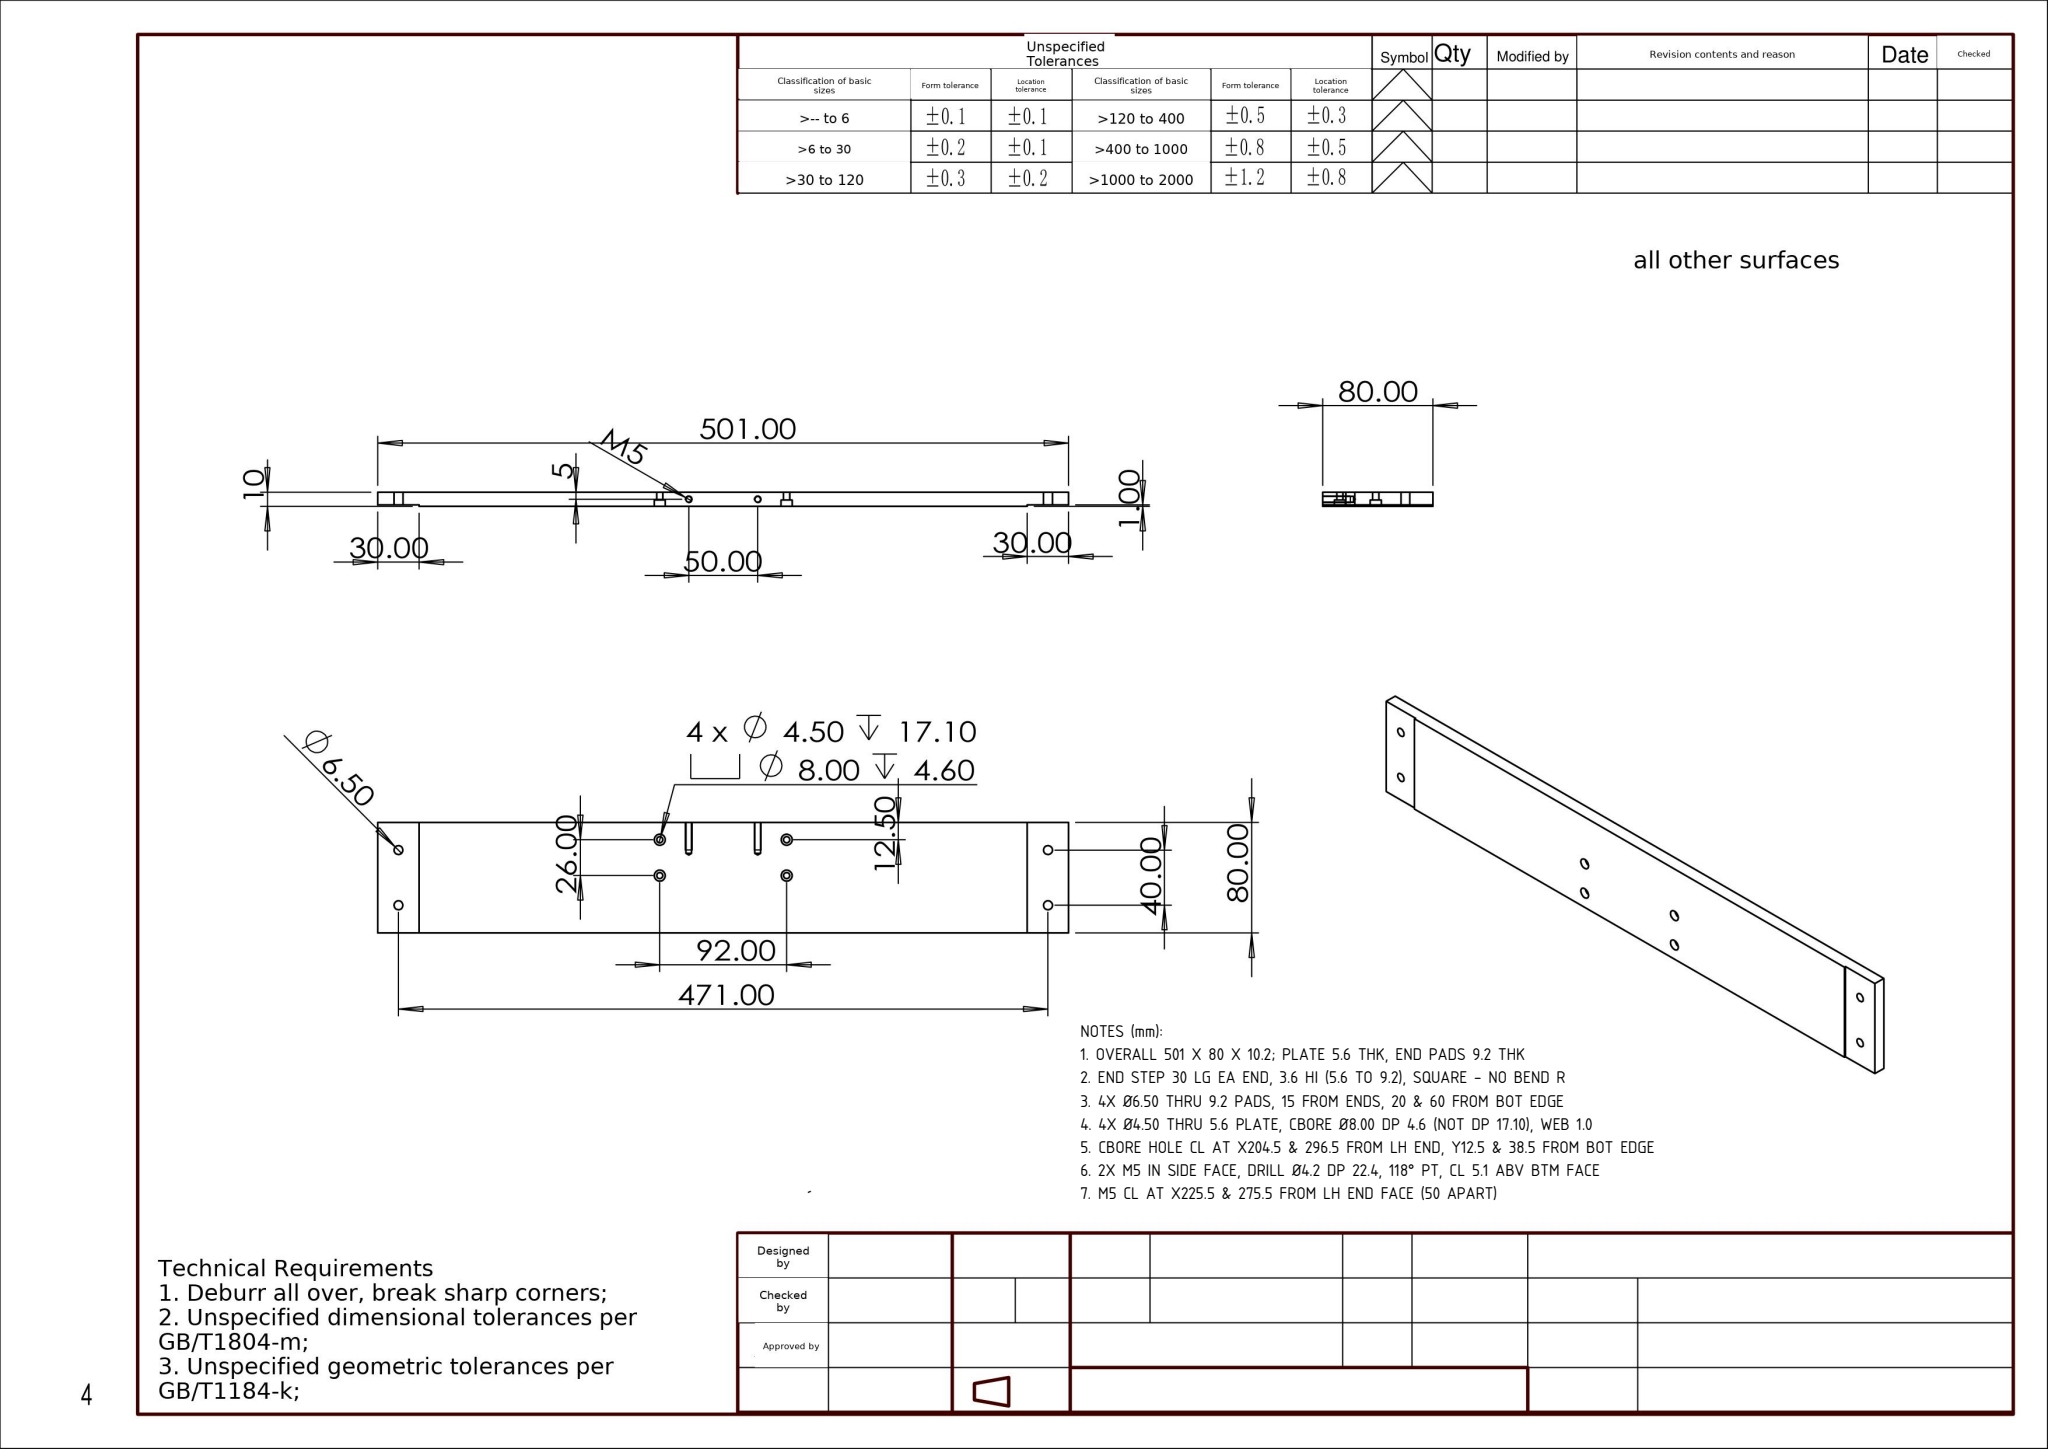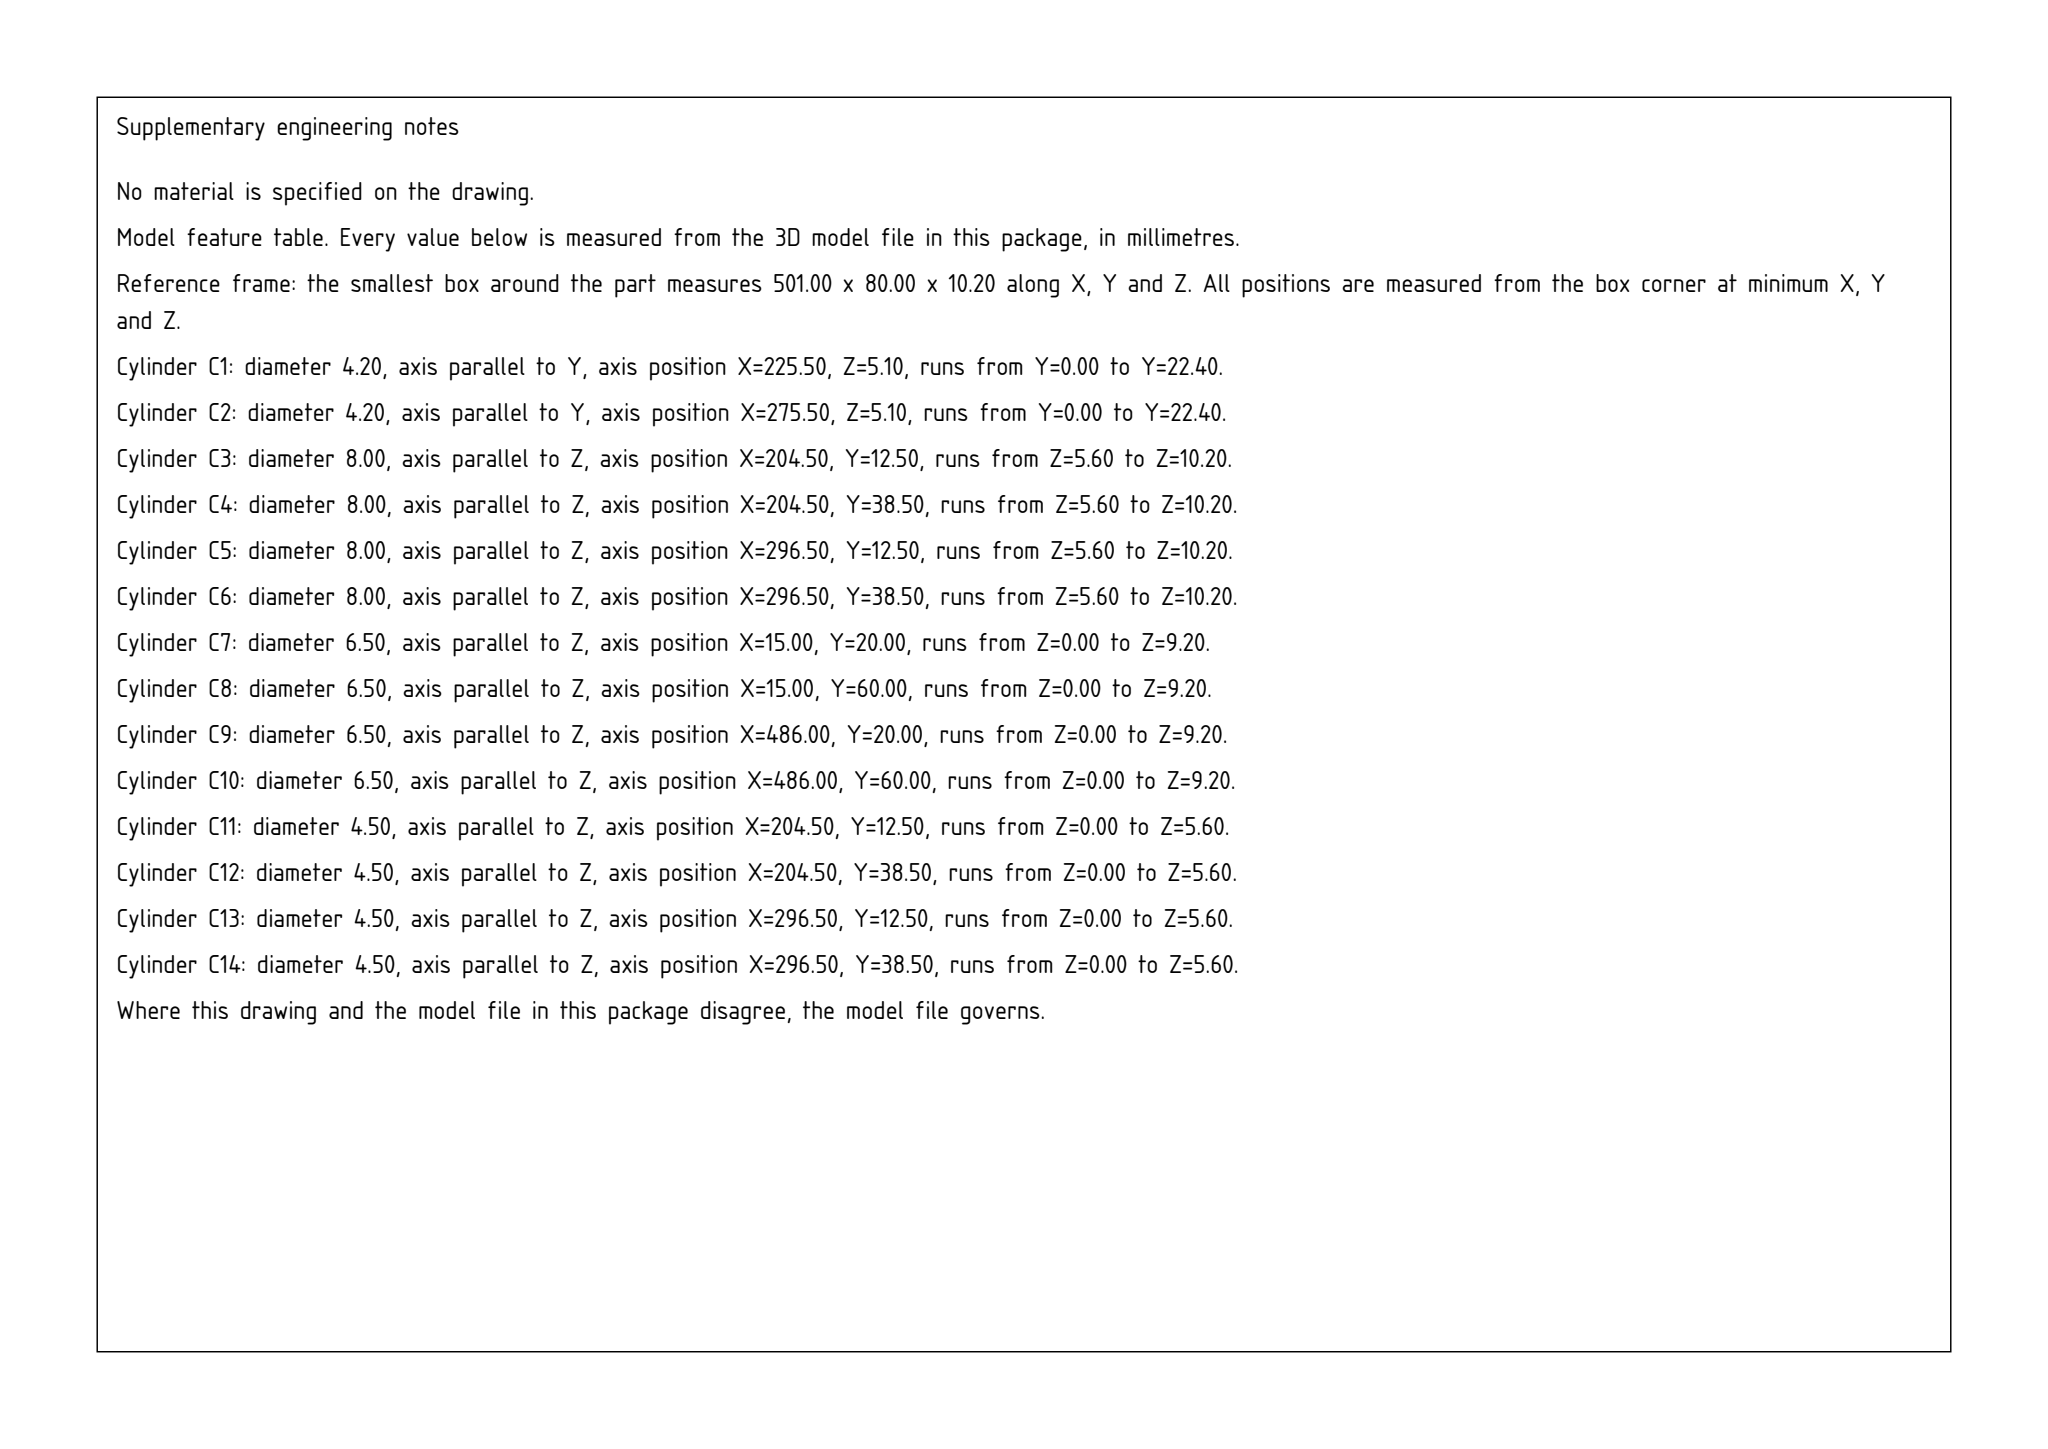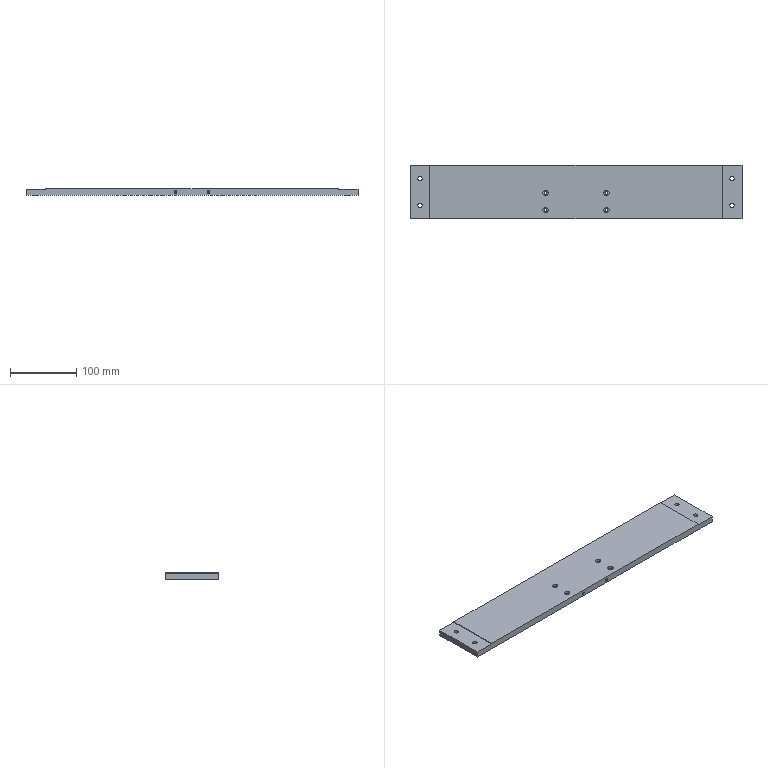Part | SolidWorks | mm | 1 solid | 46 faces | box 501 x 80 x 10.2 mm | volume 400881 mm3 | cylinder 28 | plane 14 | cone 4 | commonest cylinder face diameters 8 x8 4.5 x8 6.5 x8 4.2 x4
Drawing notes:
OVERALL 501 X 80 X 10.2; PLATE 5.6 THK, END PADS 9.2 THK | from the solid: bbox_xyz 501/80/10.2; z-planes 0, 5.6, 9.2, 10.2
END STEP 30 LG EA END, 3.6 HI (5.6 TO 9.2), SQUARE - NO BEND R | from the solid: x-planes 0/30/471/501; z 5.6 to 9.2 = 3.6; fillet_radii empty
4X Ø6.50 THRU 9.2 PADS, 15 FROM ENDS, 20 & 60 FROM BOT EDGE | from the solid: Ø6.5 z-axis cyls at (15,20),(15,60),(486,20),(486,60), len 9.2
4X Ø4.50 THRU 5.6 PLATE, CBORE Ø8.00 DP 4.6 (NOT DP 17.10), WEB 1.0 | from the solid: Ø4.5 z-cyl len 5.6 + Ø8.0 z-cyl len 4.6; 5.6-4.6=1.0 web
CBORE HOLE CL AT X204.5 & 296.5 FROM LH END, Y12.5 & 38.5 FROM BOT EDGE | from the solid: Ø4.5/Ø8.0 axes at (204.5/296.5, 12.5/38.5); 92.00 apart
2X M5 IN SIDE FACE, DRILL Ø4.2 DP 22.4, 118° PT, CL 5.1 ABV BTM FACE | from the solid: Ø4.2 y-axis cyls z=5.1, len 22.4; cone 118° ref dia 4.2
M5 CL AT X225.5 & 275.5 FROM LH END FACE (50 APART) | from the solid: Ø4.2 y-axis cyls at x=225.5 and x=275.5; bbox x=501
build123d program:
from build123d import *

# Parameters (mm, degrees)
SKETCH1_W                                         = 501
SKETCH1_H                                         = 80
BOSS_EXTRUDE1_DEPTH                               = 5.1
SKETCH2_W                                         = 30
SKETCH2_H                                         = 80
CUT_EXTRUDE1_DEPTH                                = 1
F_6_5_6_5_DIAMETER_HOLE1_D                        = 6.5
HOLE_SIZE_ACCORDING_TO_HEXAGON_SOCKET_D           = 4.5
HOLE_SIZE_ACCORDING_TO_HEXAGON_SOCKET_DEPTH       = 17.1
HOLE_SIZE_ACCORDING_TO_HEXAGON_SOCKET_CBORE_D     = 8
HOLE_SIZE_ACCORDING_TO_HEXAGON_SOCKET_CBORE_DEPTH = 4.6
HOLE_SIZE_ACCORDING_TO_HEXAGON_SOCKET_TIP         = 1.352
M5_TAPPED_HOLE1_D                                 = 4.2
M5_TAPPED_HOLE1_DEPTH                             = 22.4
M5_TAPPED_HOLE1_TIP                               = 1.262


with BuildPart() as part:
    # Sketch1 → Boss-Extrude1 (new, symmetric)
    with BuildSketch(Plane.XY):
        Rectangle(SKETCH1_W, SKETCH1_H)
    extrude(amount=BOSS_EXTRUDE1_DEPTH, both=True)

    # Sketch2 → Cut-Extrude1 (cut)
    with BuildSketch(Plane.XY.offset(5.1)):
        with Locations((-235.5, 0)):
            Rectangle(SKETCH2_W, SKETCH2_H)
    cut_extrude1 = extrude(amount=-CUT_EXTRUDE1_DEPTH, mode=Mode.SUBTRACT)

    # 6.5 _6.5_ Diameter Hole1 (through all)
    with Locations(Plane(origin=(0, 0, -5.1), x_dir=(-1, 0, 0), z_dir=(0, 0, -1))):
        with Locations((235.5, 20), (235.5, -20)):
            f_6_5_6_5_diameter_hole1 = Hole(F_6_5_6_5_DIAMETER_HOLE1_D / 2)

    # Mirror1: Cut-Extrude1, 6.5 _6.5_ Diameter Hole1 across plane
    add(cut_extrude1.mirror(Plane(origin=(0, 0, 0), x_dir=(0, 0, 1), z_dir=(1, 0, 0))), mode=Mode.SUBTRACT)
    add(f_6_5_6_5_diameter_hole1.mirror(Plane(origin=(0, 0, 0), x_dir=(0, 0, 1), z_dir=(1, 0, 0))), mode=Mode.SUBTRACT)

    # Hole Size _ according to_ Hexagon Socket
    with Locations(Plane.XY.offset(5.1)):
        with Locations((46, -1.5), (46, -27.5), (-46, -1.5), (-46, -27.5)):
            CounterBoreHole(HOLE_SIZE_ACCORDING_TO_HEXAGON_SOCKET_D / 2, HOLE_SIZE_ACCORDING_TO_HEXAGON_SOCKET_CBORE_D / 2, HOLE_SIZE_ACCORDING_TO_HEXAGON_SOCKET_CBORE_DEPTH, depth=HOLE_SIZE_ACCORDING_TO_HEXAGON_SOCKET_DEPTH)
            with Locations((0, 0, -(HOLE_SIZE_ACCORDING_TO_HEXAGON_SOCKET_DEPTH + HOLE_SIZE_ACCORDING_TO_HEXAGON_SOCKET_TIP / 2))):  # 118° drill point
                Cone(0, HOLE_SIZE_ACCORDING_TO_HEXAGON_SOCKET_D / 2, HOLE_SIZE_ACCORDING_TO_HEXAGON_SOCKET_TIP, mode=Mode.SUBTRACT)

    # M5 Tapped Hole1
    with Locations(Plane(origin=(0, -40, 0), x_dir=(-1, 0, 0), z_dir=(0, -1, 0))):
        with Locations((-25, 0), (25, 0)):
            Hole(M5_TAPPED_HOLE1_D / 2, depth=M5_TAPPED_HOLE1_DEPTH)
            with Locations((0, 0, -(M5_TAPPED_HOLE1_DEPTH + M5_TAPPED_HOLE1_TIP / 2))):  # 118° drill point
                Cone(0, M5_TAPPED_HOLE1_D / 2, M5_TAPPED_HOLE1_TIP, mode=Mode.SUBTRACT)


solid = part.part